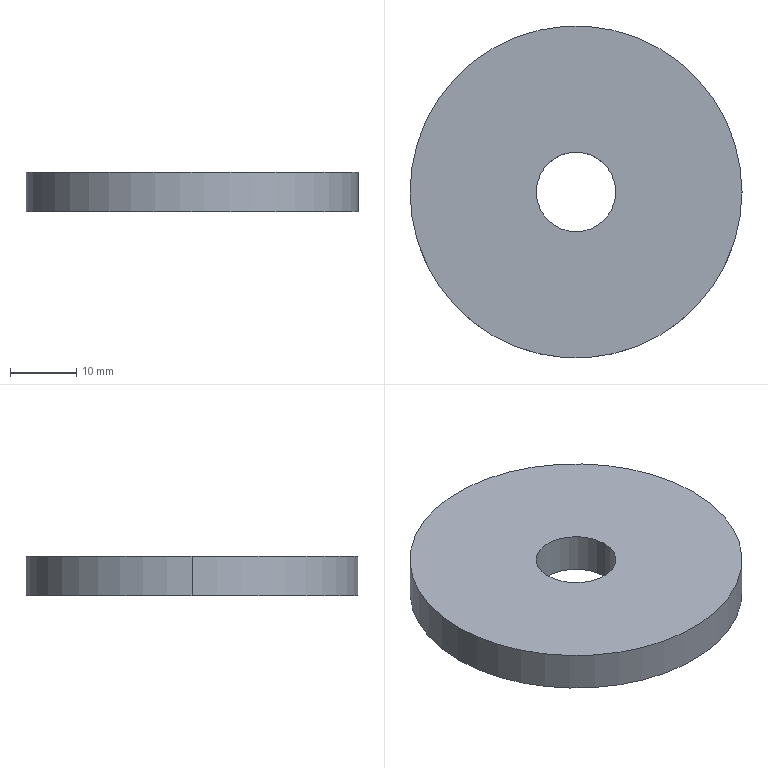Component | SolidWorks | YC1-250-03-01SliderAssembly-1_YC1-110-03-38LargeSprocketGland-1 | 1 solid | 6 faces | box 50 x 50 x 6 mm | volume 11102 mm3 | cylinder 4 | plane 2 | commonest cylinder face diameters 50 x2 12 x2 | material Plain Carbon Steel
STEP:
#1=CARTESIAN_POINT('',(9.528,88.584,-12.559));
#2=VERTEX_POINT('',#1);
#3=CARTESIAN_POINT('',(7.559,88.584,-12.559));
#4=VERTEX_POINT('',#3);
#5=CARTESIAN_POINT('',(8.543,88.584,-12.559));
#6=DIRECTION('',(0.,0.,1.));
#7=DIRECTION('',(-1.,0.,0.));
#8=AXIS2_PLACEMENT_3D('',#5,#6,#7);
#9=CIRCLE('',#8,0.9843);
#10=EDGE_CURVE('',#2,#4,#9,.T.);
#11=ORIENTED_EDGE('',*,*,#10,.F.);
#12=CARTESIAN_POINT('',(9.528,88.584,-12.795));
#13=VERTEX_POINT('',#12);
#14=CARTESIAN_POINT('',(9.528,88.584,-12.559));
#15=DIRECTION('',(0.,0.,-1.));
#16=VECTOR('',#15,39.37);
#17=LINE('',#14,#16);
#18=EDGE_CURVE('',#2,#13,#17,.T.);
#19=ORIENTED_EDGE('',*,*,#18,.T.);
#20=CARTESIAN_POINT('',(7.559,88.584,-12.795));
#21=VERTEX_POINT('',#20);
#22=CARTESIAN_POINT('',(8.543,88.584,-12.795));
#23=DIRECTION('',(0.,0.,1.));
#24=DIRECTION('',(-1.,0.,0.));
#25=AXIS2_PLACEMENT_3D('',#22,#23,#24);
#26=CIRCLE('',#25,0.9843);
#27=EDGE_CURVE('',#13,#21,#26,.T.);
#28=ORIENTED_EDGE('',*,*,#27,.T.);
#29=CARTESIAN_POINT('',(7.559,88.584,-12.559));
#30=DIRECTION('',(0.,0.,-1.));
#31=VECTOR('',#30,39.37);
#32=LINE('',#29,#31);
#33=EDGE_CURVE('',#4,#21,#32,.T.);
#34=ORIENTED_EDGE('',*,*,#33,.F.);
#35=EDGE_LOOP('',(#11,#19,#28,#34));
#36=FACE_OUTER_BOUND('',#35,.T.);
#37=CARTESIAN_POINT('',(8.543,88.584,-12.559));
#38=DIRECTION('',(0.,0.,-1.));
#39=DIRECTION('',(-1.,0.,0.));
#40=AXIS2_PLACEMENT_3D('',#37,#38,#39);
#41=CYLINDRICAL_SURFACE('',#40,0.9843);
#42=ADVANCED_FACE('',(#36),#41,.T.);
#43=CARTESIAN_POINT('',(8.307,88.584,-12.795));
#44=VERTEX_POINT('',#43);
#45=CARTESIAN_POINT('',(8.78,88.584,-12.795));
#46=VERTEX_POINT('',#45);
#47=CARTESIAN_POINT('',(8.543,88.584,-12.795));
#48=DIRECTION('',(0.,0.,1.));
#49=DIRECTION('',(1.,0.,0.));
#50=AXIS2_PLACEMENT_3D('',#47,#48,#49);
#51=CIRCLE('',#50,0.2362);
#52=EDGE_CURVE('',#44,#46,#51,.T.);
#53=ORIENTED_EDGE('',*,*,#52,.F.);
#54=CARTESIAN_POINT('',(8.307,88.584,-12.559));
#55=VERTEX_POINT('',#54);
#56=CARTESIAN_POINT('',(8.307,88.584,-12.559));
#57=DIRECTION('',(0.,0.,1.));
#58=VECTOR('',#57,39.37);
#59=LINE('',#56,#58);
#60=EDGE_CURVE('',#44,#55,#59,.T.);
#61=ORIENTED_EDGE('',*,*,#60,.T.);
#62=CARTESIAN_POINT('',(8.78,88.584,-12.559));
#63=VERTEX_POINT('',#62);
#64=CARTESIAN_POINT('',(8.543,88.584,-12.559));
#65=DIRECTION('',(0.,0.,-1.));
#66=DIRECTION('',(1.,0.,0.));
#67=AXIS2_PLACEMENT_3D('',#64,#65,#66);
#68=CIRCLE('',#67,0.2362);
#69=EDGE_CURVE('',#63,#55,#68,.T.);
#70=ORIENTED_EDGE('',*,*,#69,.F.);
#71=CARTESIAN_POINT('',(8.78,88.584,-12.559));
#72=DIRECTION('',(0.,0.,1.));
#73=VECTOR('',#72,39.37);
#74=LINE('',#71,#73);
#75=EDGE_CURVE('',#46,#63,#74,.T.);
#76=ORIENTED_EDGE('',*,*,#75,.F.);
#77=EDGE_LOOP('',(#53,#61,#70,#76));
#78=FACE_OUTER_BOUND('',#77,.T.);
#79=CARTESIAN_POINT('',(8.543,88.584,-12.559));
#80=DIRECTION('',(0.,0.,1.));
#81=DIRECTION('',(1.,0.,0.));
#82=AXIS2_PLACEMENT_3D('',#79,#80,#81);
#83=CYLINDRICAL_SURFACE('',#82,0.2362);
#84=ADVANCED_FACE('',(#78),#83,.F.);
#85=CARTESIAN_POINT('',(8.543,88.584,-12.559));
#86=DIRECTION('',(0.,0.,1.));
#87=DIRECTION('',(-1.,0.,0.));
#88=AXIS2_PLACEMENT_3D('',#85,#86,#87);
#89=CIRCLE('',#88,0.9843);
#90=EDGE_CURVE('',#4,#2,#89,.T.);
#91=ORIENTED_EDGE('',*,*,#90,.T.);
#92=ORIENTED_EDGE('',*,*,#10,.T.);
#93=EDGE_LOOP('',(#91,#92));
#94=FACE_OUTER_BOUND('',#93,.T.);
#95=ORIENTED_EDGE('',*,*,#69,.T.);
#96=CARTESIAN_POINT('',(8.543,88.584,-12.559));
#97=DIRECTION('',(0.,0.,-1.));
#98=DIRECTION('',(1.,0.,0.));
#99=AXIS2_PLACEMENT_3D('',#96,#97,#98);
#100=CIRCLE('',#99,0.2362);
#101=EDGE_CURVE('',#55,#63,#100,.T.);
#102=ORIENTED_EDGE('',*,*,#101,.T.);
#103=EDGE_LOOP('',(#95,#102));
#104=FACE_BOUND('',#103,.T.);
#105=CARTESIAN_POINT('',(8.543,88.584,-12.559));
#106=DIRECTION('',(0.,0.,1.));
#107=DIRECTION('',(1.,0.,0.));
#108=AXIS2_PLACEMENT_3D('',#105,#106,#107);
#109=PLANE('',#108);
#110=ADVANCED_FACE('',(#94,#104),#109,.T.);
#111=ORIENTED_EDGE('',*,*,#18,.F.);
#112=ORIENTED_EDGE('',*,*,#90,.F.);
#113=ORIENTED_EDGE('',*,*,#33,.T.);
#114=CARTESIAN_POINT('',(8.543,88.584,-12.795));
#115=DIRECTION('',(0.,0.,1.));
#116=DIRECTION('',(-1.,0.,0.));
#117=AXIS2_PLACEMENT_3D('',#114,#115,#116);
#118=CIRCLE('',#117,0.9843);
#119=EDGE_CURVE('',#21,#13,#118,.T.);
#120=ORIENTED_EDGE('',*,*,#119,.T.);
#121=EDGE_LOOP('',(#111,#112,#113,#120));
#122=FACE_OUTER_BOUND('',#121,.T.);
#123=CARTESIAN_POINT('',(8.543,88.584,-12.559));
#124=DIRECTION('',(0.,0.,-1.));
#125=DIRECTION('',(-1.,0.,0.));
#126=AXIS2_PLACEMENT_3D('',#123,#124,#125);
#127=CYLINDRICAL_SURFACE('',#126,0.9843);
#128=ADVANCED_FACE('',(#122),#127,.T.);
#129=ORIENTED_EDGE('',*,*,#60,.F.);
#130=CARTESIAN_POINT('',(8.543,88.584,-12.795));
#131=DIRECTION('',(0.,0.,1.));
#132=DIRECTION('',(1.,0.,0.));
#133=AXIS2_PLACEMENT_3D('',#130,#131,#132);
#134=CIRCLE('',#133,0.2362);
#135=EDGE_CURVE('',#46,#44,#134,.T.);
#136=ORIENTED_EDGE('',*,*,#135,.F.);
#137=ORIENTED_EDGE('',*,*,#75,.T.);
#138=ORIENTED_EDGE('',*,*,#101,.F.);
#139=EDGE_LOOP('',(#129,#136,#137,#138));
#140=FACE_OUTER_BOUND('',#139,.T.);
#141=CARTESIAN_POINT('',(8.543,88.584,-12.559));
#142=DIRECTION('',(0.,0.,1.));
#143=DIRECTION('',(1.,0.,0.));
#144=AXIS2_PLACEMENT_3D('',#141,#142,#143);
#145=CYLINDRICAL_SURFACE('',#144,0.2362);
#146=ADVANCED_FACE('',(#140),#145,.F.);
#147=ORIENTED_EDGE('',*,*,#119,.F.);
#148=ORIENTED_EDGE('',*,*,#27,.F.);
#149=EDGE_LOOP('',(#147,#148));
#150=FACE_OUTER_BOUND('',#149,.T.);
#151=ORIENTED_EDGE('',*,*,#135,.T.);
#152=ORIENTED_EDGE('',*,*,#52,.T.);
#153=EDGE_LOOP('',(#151,#152));
#154=FACE_BOUND('',#153,.T.);
#155=CARTESIAN_POINT('',(8.543,88.584,-12.795));
#156=DIRECTION('',(0.,0.,1.));
#157=DIRECTION('',(1.,0.,0.));
#158=AXIS2_PLACEMENT_3D('',#155,#156,#157);
#159=PLANE('',#158);
#160=ADVANCED_FACE('',(#150,#154),#159,.F.);
#161=CLOSED_SHELL('',(#42,#84,#110,#128,#146,#160));
#162=MANIFOLD_SOLID_BREP('',#161);
#163=CARTESIAN_POINT('',(0.,0.,0.));
#164=DIRECTION('',(0.,0.,1.));
#165=DIRECTION('',(1.,0.,0.));
#166=AXIS2_PLACEMENT_3D('',#163,#164,#165);
#167=(LENGTH_UNIT()NAMED_UNIT(*)SI_UNIT($,.METRE.));
#168=LENGTH_MEASURE_WITH_UNIT(LENGTH_MEASURE(0.0254),#167);
#169=DIMENSIONAL_EXPONENTS(1.,0.,0.,0.,0.,0.,0.);
#170=(CONVERSION_BASED_UNIT('',#168)LENGTH_UNIT()NAMED_UNIT(#169));
#171=UNCERTAINTY_MEASURE_WITH_UNIT(LENGTH_MEASURE(0.00001),#170,'','');
#172=(NAMED_UNIT(*)PLANE_ANGLE_UNIT()SI_UNIT($,.RADIAN.));
#173=(NAMED_UNIT(*)SI_UNIT($,.STERADIAN.)SOLID_ANGLE_UNIT());
#174=(GEOMETRIC_REPRESENTATION_CONTEXT(3)GLOBAL_UNCERTAINTY_ASSIGNED_CONTEXT((#171))GLOBAL_UNIT_ASSIGNED_CONTEXT((#170,#172,#173))REPRESENTATION_CONTEXT('',''));
#175=ADVANCED_BREP_SHAPE_REPRESENTATION('',(#162,#166),#174);
#176=COLOUR_RGB('',0.7922,0.8196,0.9333);
#177=FILL_AREA_STYLE_COLOUR('',#176);
#178=FILL_AREA_STYLE('',(#177));
#179=SURFACE_STYLE_FILL_AREA(#178);
#180=SURFACE_SIDE_STYLE('',(#179));
#181=SURFACE_STYLE_USAGE(.BOTH.,#180);
#182=PRESENTATION_STYLE_ASSIGNMENT((#181));
#183=STYLED_ITEM('',(#182),#162);
#184=PRESENTATION_LAYER_ASSIGNMENT('','',(#183));
#185=(LENGTH_UNIT()NAMED_UNIT(*)SI_UNIT($,.METRE.));
#186=LENGTH_MEASURE_WITH_UNIT(LENGTH_MEASURE(0.0254),#185);
#187=DIMENSIONAL_EXPONENTS(1.,0.,0.,0.,0.,0.,0.);
#188=(CONVERSION_BASED_UNIT('',#186)LENGTH_UNIT()NAMED_UNIT(#187));
#189=UNCERTAINTY_MEASURE_WITH_UNIT(LENGTH_MEASURE(0.00001),#188,'','');
#190=(NAMED_UNIT(*)PLANE_ANGLE_UNIT()SI_UNIT($,.RADIAN.));
#191=(NAMED_UNIT(*)SI_UNIT($,.STERADIAN.)SOLID_ANGLE_UNIT());
#192=(GEOMETRIC_REPRESENTATION_CONTEXT(3)GLOBAL_UNCERTAINTY_ASSIGNED_CONTEXT((#189))GLOBAL_UNIT_ASSIGNED_CONTEXT((#188,#190,#191))REPRESENTATION_CONTEXT('',''));
#193=MECHANICAL_DESIGN_GEOMETRIC_PRESENTATION_REPRESENTATION('',(#183),#192);